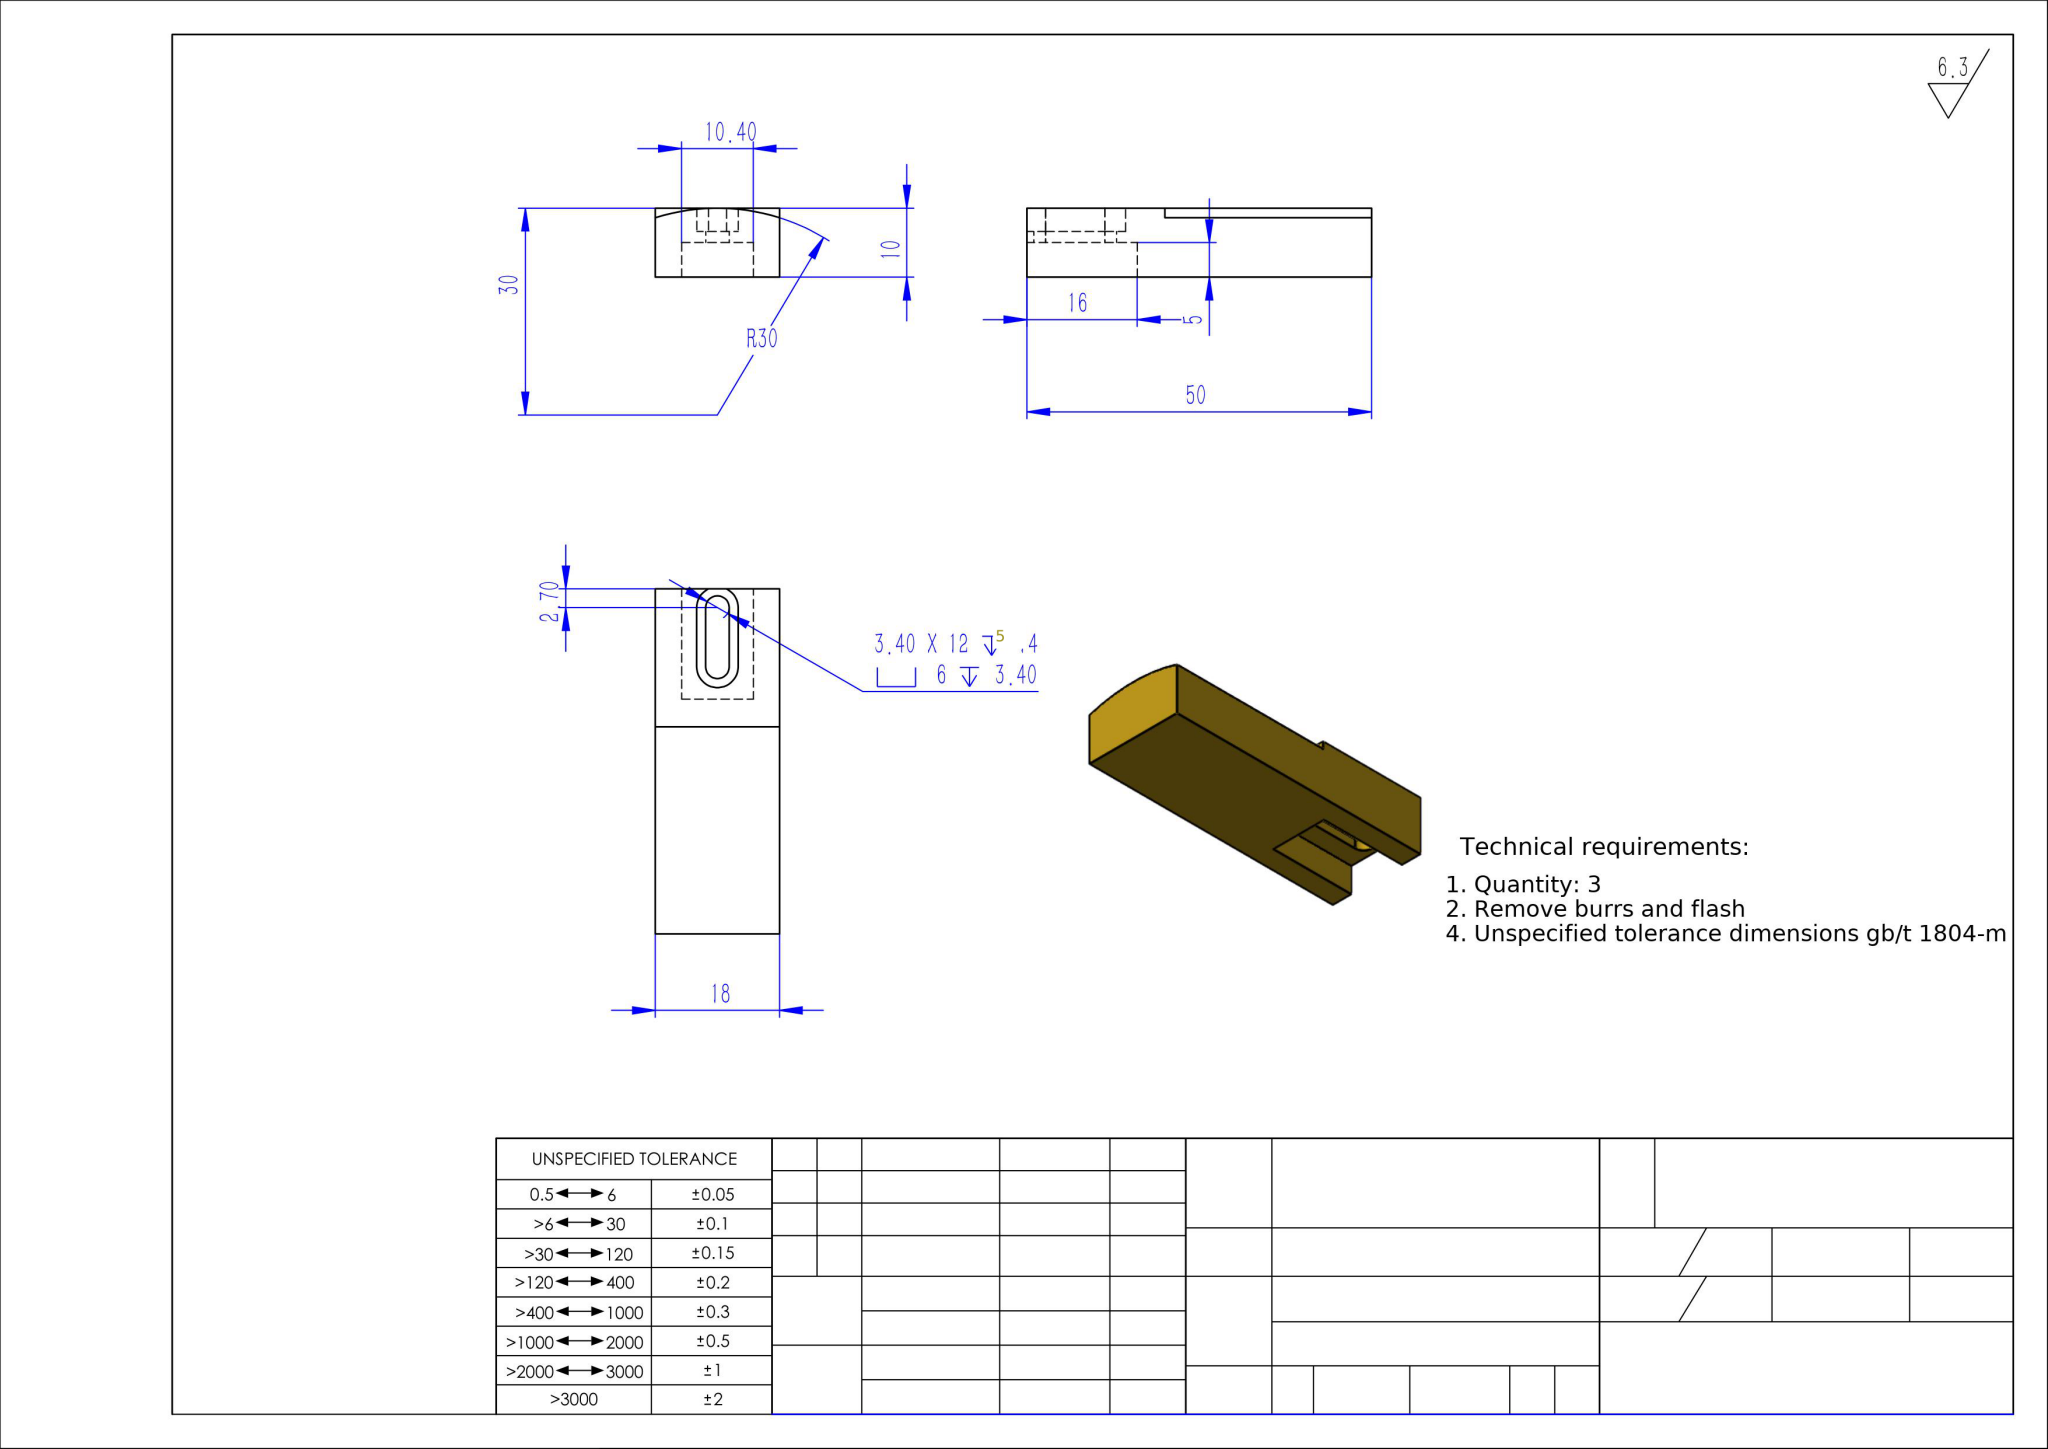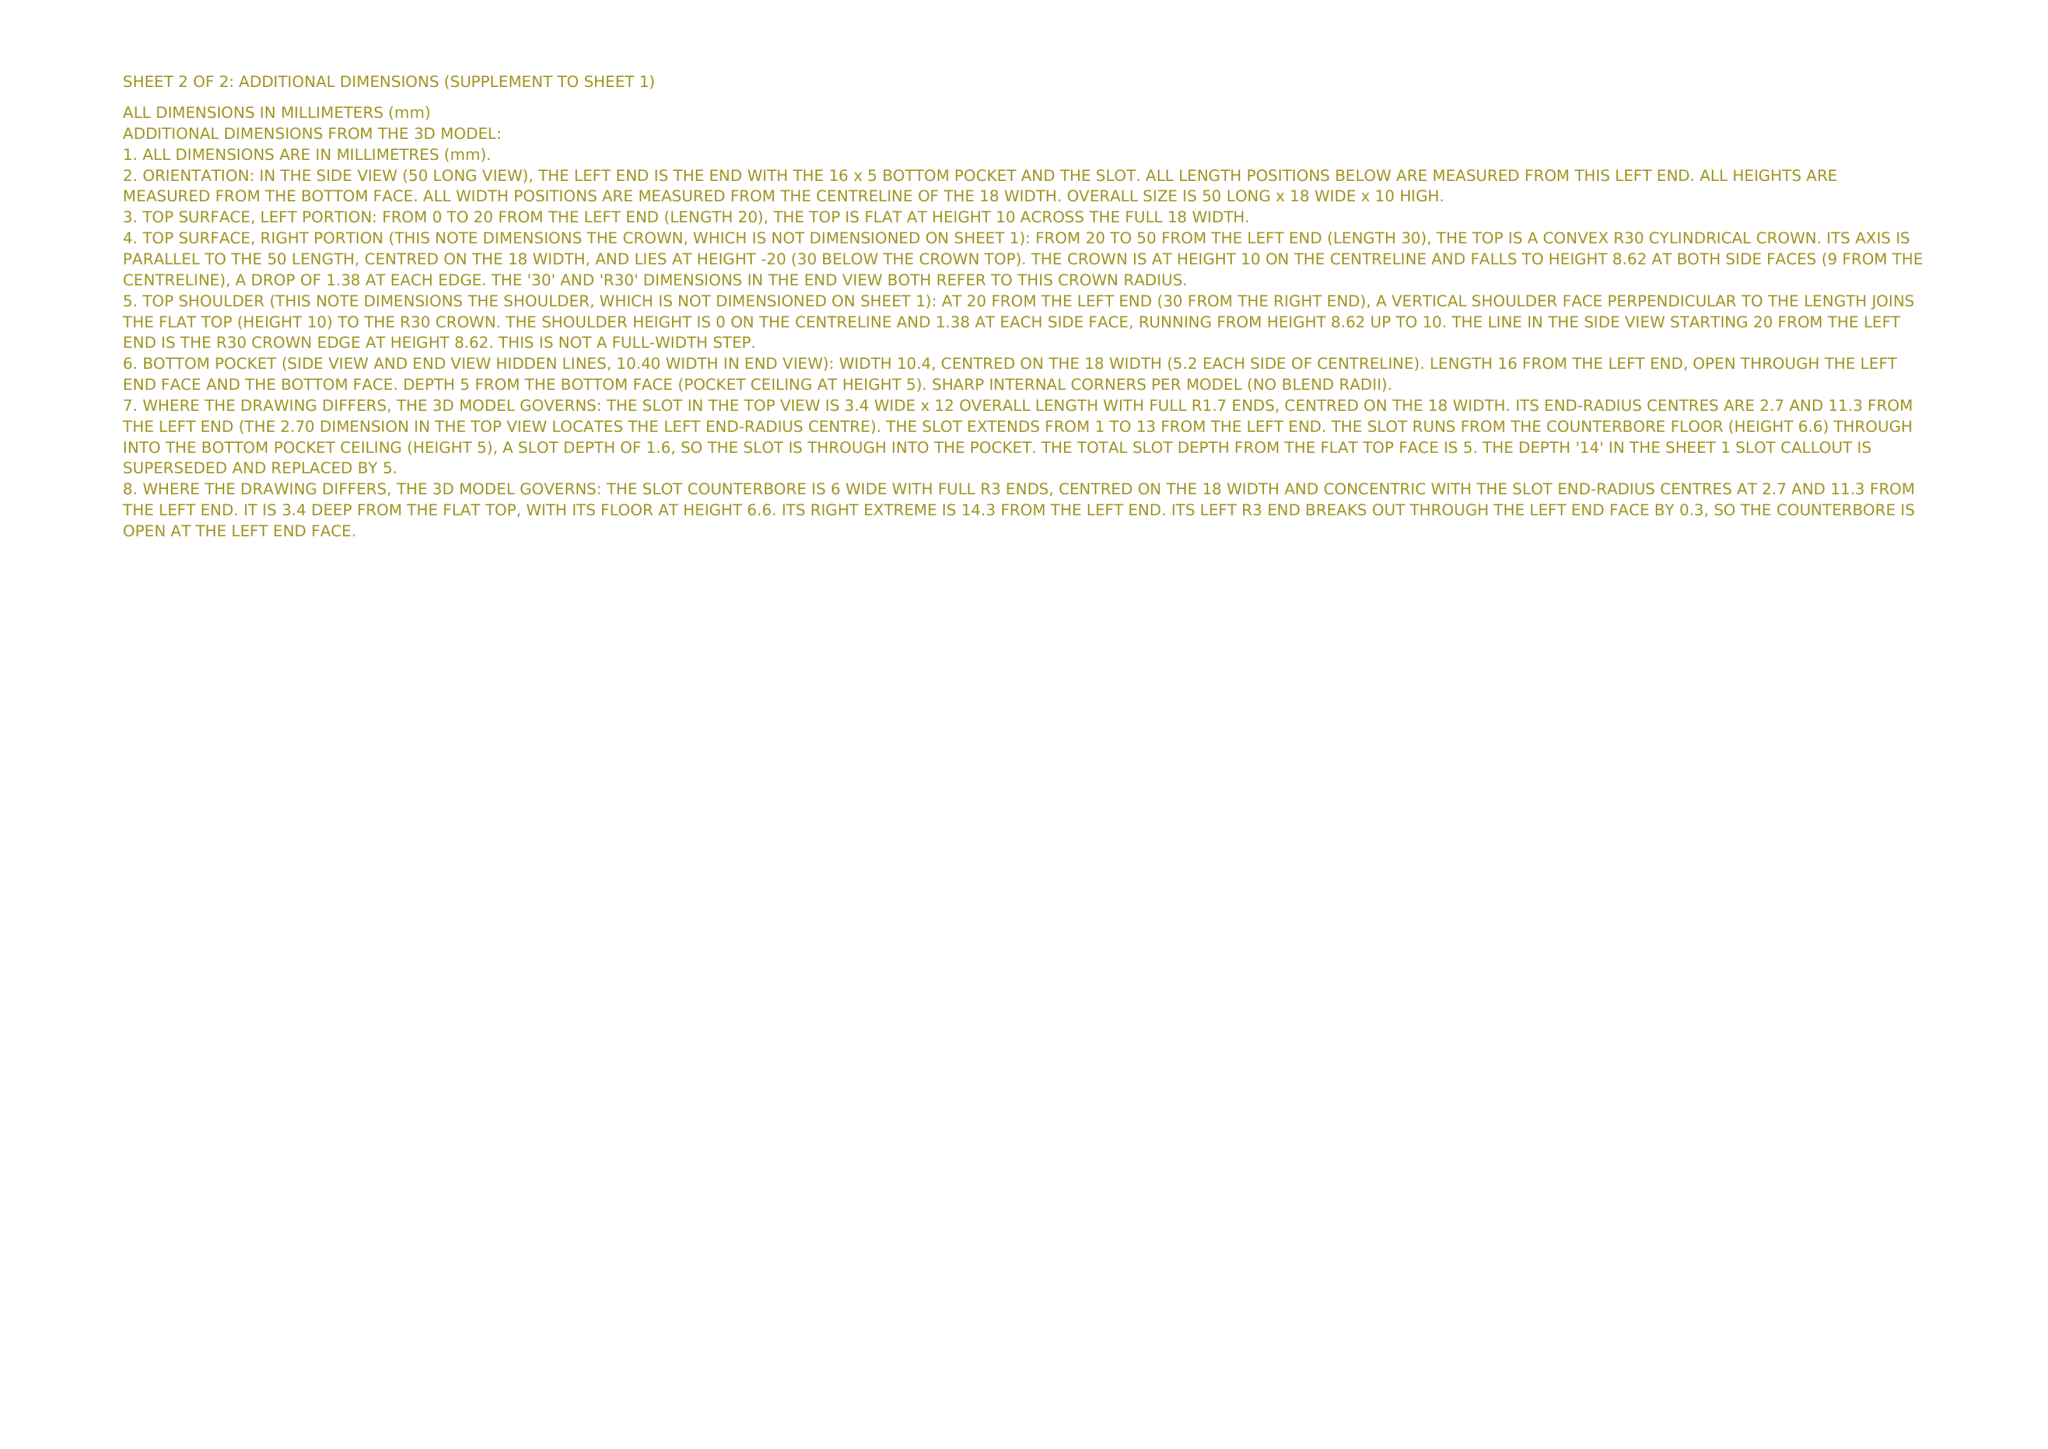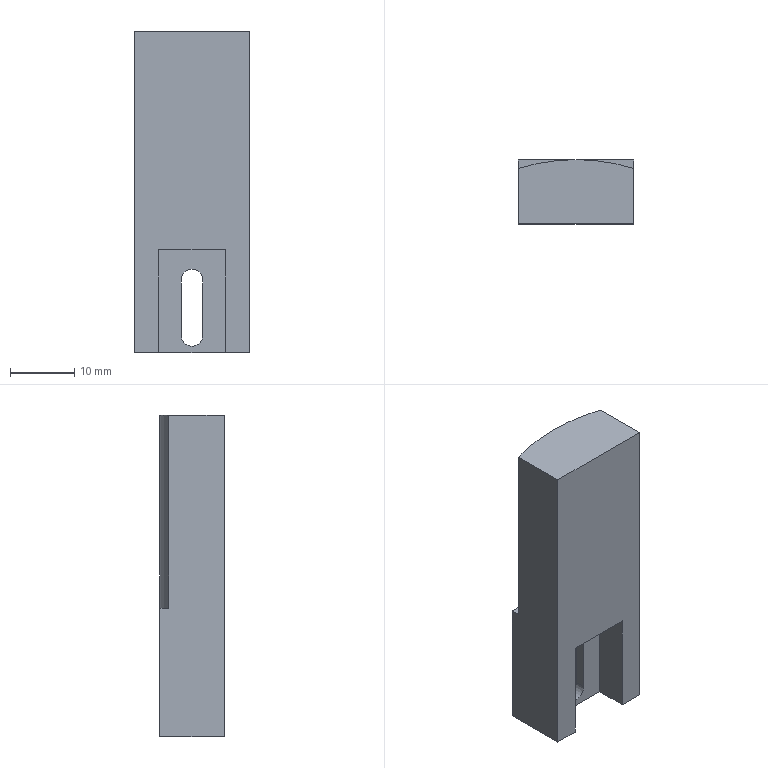Part | NX | mm | Stepped L-Shaped Slotted Mounting Bracket | 1 solid | 25 faces | box 18 x 10 x 50 mm | volume 7591 mm3 | plane 17 | cylinder 8 | commonest cylinder face diameters 6 x4 3.4 x3 60 x1
STEP:
#1=COLOUR_RGB('',0.6471,0.5176,0.);
#2=FILL_AREA_STYLE_COLOUR('',#1);
#3=FILL_AREA_STYLE('',(#2));
#4=SURFACE_STYLE_FILL_AREA(#3);
#5=SURFACE_SIDE_STYLE('',(#4));
#6=SURFACE_STYLE_USAGE(.BOTH.,#5);
#7=PRESENTATION_STYLE_ASSIGNMENT((#6));
#8=CARTESIAN_POINT('',(0.,6.6,-10.7));
#9=VERTEX_POINT('',#8);
#10=CARTESIAN_POINT('',(3.,6.6,-13.7));
#11=VERTEX_POINT('',#10);
#12=CARTESIAN_POINT('',(0.,6.6,-13.7));
#13=DIRECTION('',(0.,1.,0.));
#14=DIRECTION('',(0.,0.,1.));
#15=AXIS2_PLACEMENT_3D('',#12,#13,#14);
#16=CIRCLE('',#15,3.);
#17=EDGE_CURVE('',#9,#11,#16,.T.);
#18=ORIENTED_EDGE('',*,*,#17,.F.);
#19=CARTESIAN_POINT('',(0.,10.,-10.7));
#20=VERTEX_POINT('',#19);
#21=CARTESIAN_POINT('',(0.,10.,-10.7));
#22=DIRECTION('',(0.,1.,0.));
#23=VECTOR('',#22,1000.);
#24=LINE('',#21,#23);
#25=EDGE_CURVE('',#9,#20,#24,.T.);
#26=ORIENTED_EDGE('',*,*,#25,.T.);
#27=CARTESIAN_POINT('',(3.,10.,-13.7));
#28=VERTEX_POINT('',#27);
#29=CARTESIAN_POINT('',(0.,10.,-13.7));
#30=DIRECTION('',(0.,1.,0.));
#31=DIRECTION('',(0.,0.,1.));
#32=AXIS2_PLACEMENT_3D('',#29,#30,#31);
#33=CIRCLE('',#32,3.);
#34=EDGE_CURVE('',#20,#28,#33,.T.);
#35=ORIENTED_EDGE('',*,*,#34,.T.);
#36=CARTESIAN_POINT('',(3.,6.6,-13.7));
#37=DIRECTION('',(-0.,-1.,0.));
#38=VECTOR('',#37,1000.);
#39=LINE('',#36,#38);
#40=EDGE_CURVE('',#28,#11,#39,.T.);
#41=ORIENTED_EDGE('',*,*,#40,.T.);
#42=EDGE_LOOP('',(#18,#26,#35,#41));
#43=FACE_OUTER_BOUND('',#42,.T.);
#44=CARTESIAN_POINT('',(0.,10.,-13.7));
#45=DIRECTION('',(0.,1.,0.));
#46=DIRECTION('',(0.,0.,1.));
#47=AXIS2_PLACEMENT_3D('',#44,#45,#46);
#48=CYLINDRICAL_SURFACE('',#47,3.);
#49=ADVANCED_FACE('',(#43),#48,.F.);
#50=CARTESIAN_POINT('',(1.7,5.,-13.7));
#51=VERTEX_POINT('',#50);
#52=CARTESIAN_POINT('',(0.,5.,-12.));
#53=VERTEX_POINT('',#52);
#54=CARTESIAN_POINT('',(0.,5.,-13.7));
#55=DIRECTION('',(0.,-1.,0.));
#56=DIRECTION('',(0.,0.,1.));
#57=AXIS2_PLACEMENT_3D('',#54,#55,#56);
#58=CIRCLE('',#57,1.7);
#59=EDGE_CURVE('',#51,#53,#58,.T.);
#60=ORIENTED_EDGE('',*,*,#59,.T.);
#61=CARTESIAN_POINT('',(0.,6.6,-12.));
#62=VERTEX_POINT('',#61);
#63=CARTESIAN_POINT('',(0.,10.,-12.));
#64=DIRECTION('',(0.,1.,0.));
#65=VECTOR('',#64,1000.);
#66=LINE('',#63,#65);
#67=EDGE_CURVE('',#53,#62,#66,.T.);
#68=ORIENTED_EDGE('',*,*,#67,.T.);
#69=CARTESIAN_POINT('',(1.7,6.6,-13.7));
#70=VERTEX_POINT('',#69);
#71=CARTESIAN_POINT('',(0.,6.6,-13.7));
#72=DIRECTION('',(0.,1.,0.));
#73=DIRECTION('',(0.,0.,1.));
#74=AXIS2_PLACEMENT_3D('',#71,#72,#73);
#75=CIRCLE('',#74,1.7);
#76=EDGE_CURVE('',#62,#70,#75,.T.);
#77=ORIENTED_EDGE('',*,*,#76,.T.);
#78=CARTESIAN_POINT('',(1.7,-4.,-13.7));
#79=DIRECTION('',(-0.,-1.,0.));
#80=VECTOR('',#79,1000.);
#81=LINE('',#78,#80);
#82=EDGE_CURVE('',#70,#51,#81,.T.);
#83=ORIENTED_EDGE('',*,*,#82,.T.);
#84=EDGE_LOOP('',(#60,#68,#77,#83));
#85=FACE_OUTER_BOUND('',#84,.T.);
#86=CARTESIAN_POINT('',(0.,10.,-13.7));
#87=DIRECTION('',(0.,1.,0.));
#88=DIRECTION('',(0.,0.,1.));
#89=AXIS2_PLACEMENT_3D('',#86,#87,#88);
#90=CYLINDRICAL_SURFACE('',#89,1.7);
#91=ADVANCED_FACE('',(#85),#90,.F.);
#92=CARTESIAN_POINT('',(9.,8.618,25.));
#93=VERTEX_POINT('',#92);
#94=CARTESIAN_POINT('',(9.,0.,25.));
#95=VERTEX_POINT('',#94);
#96=CARTESIAN_POINT('',(9.,10.,25.));
#97=DIRECTION('',(0.,-1.,0.));
#98=VECTOR('',#97,1000.);
#99=LINE('',#96,#98);
#100=EDGE_CURVE('',#93,#95,#99,.T.);
#101=ORIENTED_EDGE('',*,*,#100,.F.);
#102=CARTESIAN_POINT('',(-9.,8.618,25.));
#103=VERTEX_POINT('',#102);
#104=CARTESIAN_POINT('',(0.,-20.,25.));
#105=DIRECTION('',(0.,0.,1.));
#106=DIRECTION('',(1.,0.,0.));
#107=AXIS2_PLACEMENT_3D('',#104,#105,#106);
#108=CIRCLE('',#107,30.);
#109=EDGE_CURVE('',#93,#103,#108,.T.);
#110=ORIENTED_EDGE('',*,*,#109,.T.);
#111=CARTESIAN_POINT('',(-9.,0.,25.));
#112=VERTEX_POINT('',#111);
#113=CARTESIAN_POINT('',(-9.,10.,25.));
#114=DIRECTION('',(0.,-1.,0.));
#115=VECTOR('',#114,1000.);
#116=LINE('',#113,#115);
#117=EDGE_CURVE('',#103,#112,#116,.T.);
#118=ORIENTED_EDGE('',*,*,#117,.T.);
#119=CARTESIAN_POINT('',(-9.,0.,25.));
#120=DIRECTION('',(1.,0.,0.));
#121=VECTOR('',#120,1000.);
#122=LINE('',#119,#121);
#123=EDGE_CURVE('',#112,#95,#122,.T.);
#124=ORIENTED_EDGE('',*,*,#123,.T.);
#125=EDGE_LOOP('',(#101,#110,#118,#124));
#126=FACE_OUTER_BOUND('',#125,.T.);
#127=CARTESIAN_POINT('',(-9.,10.,25.));
#128=DIRECTION('',(0.,0.,-1.));
#129=DIRECTION('',(-1.,0.,0.));
#130=AXIS2_PLACEMENT_3D('',#127,#128,#129);
#131=PLANE('',#130);
#132=ADVANCED_FACE('',(#126),#131,.F.);
#133=CARTESIAN_POINT('',(0.,10.,-5.));
#134=VERTEX_POINT('',#133);
#135=CARTESIAN_POINT('',(-9.,10.,-5.));
#136=VERTEX_POINT('',#135);
#137=CARTESIAN_POINT('',(0.,10.,-5.));
#138=DIRECTION('',(-1.,0.,0.));
#139=VECTOR('',#138,1000.);
#140=LINE('',#137,#139);
#141=EDGE_CURVE('',#134,#136,#140,.T.);
#142=ORIENTED_EDGE('',*,*,#141,.F.);
#143=CARTESIAN_POINT('',(9.,10.,-5.));
#144=VERTEX_POINT('',#143);
#145=CARTESIAN_POINT('',(0.,10.,-5.));
#146=DIRECTION('',(-1.,0.,0.));
#147=VECTOR('',#146,1000.);
#148=LINE('',#145,#147);
#149=EDGE_CURVE('',#144,#134,#148,.T.);
#150=ORIENTED_EDGE('',*,*,#149,.F.);
#151=CARTESIAN_POINT('',(9.,10.,-25.));
#152=VERTEX_POINT('',#151);
#153=CARTESIAN_POINT('',(9.,10.,-25.));
#154=DIRECTION('',(-0.,0.,-1.));
#155=VECTOR('',#154,1000.);
#156=LINE('',#153,#155);
#157=EDGE_CURVE('',#144,#152,#156,.T.);
#158=ORIENTED_EDGE('',*,*,#157,.T.);
#159=CARTESIAN_POINT('',(1.308,10.,-25.));
#160=VERTEX_POINT('',#159);
#161=CARTESIAN_POINT('',(-9.,10.,-25.));
#162=DIRECTION('',(-1.,0.,0.));
#163=VECTOR('',#162,1000.);
#164=LINE('',#161,#163);
#165=EDGE_CURVE('',#152,#160,#164,.T.);
#166=ORIENTED_EDGE('',*,*,#165,.T.);
#167=CARTESIAN_POINT('',(3.,10.,-22.3));
#168=VERTEX_POINT('',#167);
#169=CARTESIAN_POINT('',(0.,10.,-22.3));
#170=DIRECTION('',(0.,1.,0.));
#171=DIRECTION('',(0.,0.,1.));
#172=AXIS2_PLACEMENT_3D('',#169,#170,#171);
#173=CIRCLE('',#172,3.);
#174=EDGE_CURVE('',#168,#160,#173,.T.);
#175=ORIENTED_EDGE('',*,*,#174,.F.);
#176=CARTESIAN_POINT('',(3.,10.,-22.3));
#177=DIRECTION('',(0.,0.,1.));
#178=VECTOR('',#177,1000.);
#179=LINE('',#176,#178);
#180=EDGE_CURVE('',#168,#28,#179,.T.);
#181=ORIENTED_EDGE('',*,*,#180,.T.);
#182=ORIENTED_EDGE('',*,*,#34,.F.);
#183=CARTESIAN_POINT('',(-3.,10.,-13.7));
#184=VERTEX_POINT('',#183);
#185=CARTESIAN_POINT('',(0.,10.,-13.7));
#186=DIRECTION('',(0.,1.,0.));
#187=DIRECTION('',(0.,0.,1.));
#188=AXIS2_PLACEMENT_3D('',#185,#186,#187);
#189=CIRCLE('',#188,3.);
#190=EDGE_CURVE('',#184,#20,#189,.T.);
#191=ORIENTED_EDGE('',*,*,#190,.F.);
#192=CARTESIAN_POINT('',(-3.,10.,-22.3));
#193=VERTEX_POINT('',#192);
#194=CARTESIAN_POINT('',(-3.,10.,-22.3));
#195=DIRECTION('',(0.,0.,1.));
#196=VECTOR('',#195,1000.);
#197=LINE('',#194,#196);
#198=EDGE_CURVE('',#193,#184,#197,.T.);
#199=ORIENTED_EDGE('',*,*,#198,.F.);
#200=CARTESIAN_POINT('',(-1.308,10.,-25.));
#201=VERTEX_POINT('',#200);
#202=CARTESIAN_POINT('',(0.,10.,-22.3));
#203=DIRECTION('',(0.,1.,0.));
#204=DIRECTION('',(0.,0.,1.));
#205=AXIS2_PLACEMENT_3D('',#202,#203,#204);
#206=CIRCLE('',#205,3.);
#207=EDGE_CURVE('',#201,#193,#206,.T.);
#208=ORIENTED_EDGE('',*,*,#207,.F.);
#209=CARTESIAN_POINT('',(-9.,10.,-25.));
#210=VERTEX_POINT('',#209);
#211=CARTESIAN_POINT('',(-9.,10.,-25.));
#212=DIRECTION('',(-1.,0.,0.));
#213=VECTOR('',#212,1000.);
#214=LINE('',#211,#213);
#215=EDGE_CURVE('',#201,#210,#214,.T.);
#216=ORIENTED_EDGE('',*,*,#215,.T.);
#217=CARTESIAN_POINT('',(-9.,10.,-25.));
#218=DIRECTION('',(0.,0.,1.));
#219=VECTOR('',#218,1000.);
#220=LINE('',#217,#219);
#221=EDGE_CURVE('',#210,#136,#220,.T.);
#222=ORIENTED_EDGE('',*,*,#221,.T.);
#223=EDGE_LOOP('',(#142,#150,#158,#166,#175,#181,#182,#191,#199,#208,#216,#222));
#224=FACE_OUTER_BOUND('',#223,.T.);
#225=CARTESIAN_POINT('',(0.,10.,0.));
#226=DIRECTION('',(0.,1.,0.));
#227=DIRECTION('',(0.,0.,1.));
#228=AXIS2_PLACEMENT_3D('',#225,#226,#227);
#229=PLANE('',#228);
#230=ADVANCED_FACE('',(#224),#229,.T.);
#231=CARTESIAN_POINT('',(9.,8.618,-5.));
#232=VERTEX_POINT('',#231);
#233=CARTESIAN_POINT('',(9.,8.618,-5.));
#234=DIRECTION('',(0.,0.,1.));
#235=VECTOR('',#234,1000.);
#236=LINE('',#233,#235);
#237=EDGE_CURVE('',#232,#93,#236,.T.);
#238=ORIENTED_EDGE('',*,*,#237,.T.);
#239=ORIENTED_EDGE('',*,*,#100,.T.);
#240=CARTESIAN_POINT('',(9.,0.,-25.));
#241=VERTEX_POINT('',#240);
#242=CARTESIAN_POINT('',(9.,0.,-25.));
#243=DIRECTION('',(-0.,0.,-1.));
#244=VECTOR('',#243,1000.);
#245=LINE('',#242,#244);
#246=EDGE_CURVE('',#95,#241,#245,.T.);
#247=ORIENTED_EDGE('',*,*,#246,.T.);
#248=CARTESIAN_POINT('',(9.,10.,-25.));
#249=DIRECTION('',(0.,-1.,0.));
#250=VECTOR('',#249,1000.);
#251=LINE('',#248,#250);
#252=EDGE_CURVE('',#152,#241,#251,.T.);
#253=ORIENTED_EDGE('',*,*,#252,.F.);
#254=ORIENTED_EDGE('',*,*,#157,.F.);
#255=CARTESIAN_POINT('',(9.,0.,-5.));
#256=DIRECTION('',(0.,1.,0.));
#257=VECTOR('',#256,1000.);
#258=LINE('',#255,#257);
#259=EDGE_CURVE('',#232,#144,#258,.T.);
#260=ORIENTED_EDGE('',*,*,#259,.F.);
#261=EDGE_LOOP('',(#238,#239,#247,#253,#254,#260));
#262=FACE_OUTER_BOUND('',#261,.T.);
#263=CARTESIAN_POINT('',(9.,10.,-25.));
#264=DIRECTION('',(-1.,0.,0.));
#265=DIRECTION('',(0.,0.,1.));
#266=AXIS2_PLACEMENT_3D('',#263,#264,#265);
#267=PLANE('',#266);
#268=ADVANCED_FACE('',(#262),#267,.F.);
#269=CARTESIAN_POINT('',(-9.,8.618,-5.));
#270=VERTEX_POINT('',#269);
#271=CARTESIAN_POINT('',(-9.,8.618,-5.));
#272=DIRECTION('',(0.,0.,1.));
#273=VECTOR('',#272,1000.);
#274=LINE('',#271,#273);
#275=EDGE_CURVE('',#270,#103,#274,.T.);
#276=ORIENTED_EDGE('',*,*,#275,.F.);
#277=CARTESIAN_POINT('',(-9.,0.,-5.));
#278=DIRECTION('',(0.,-1.,0.));
#279=VECTOR('',#278,1000.);
#280=LINE('',#277,#279);
#281=EDGE_CURVE('',#136,#270,#280,.T.);
#282=ORIENTED_EDGE('',*,*,#281,.F.);
#283=ORIENTED_EDGE('',*,*,#221,.F.);
#284=CARTESIAN_POINT('',(-9.,0.,-25.));
#285=VERTEX_POINT('',#284);
#286=CARTESIAN_POINT('',(-9.,10.,-25.));
#287=DIRECTION('',(0.,-1.,0.));
#288=VECTOR('',#287,1000.);
#289=LINE('',#286,#288);
#290=EDGE_CURVE('',#210,#285,#289,.T.);
#291=ORIENTED_EDGE('',*,*,#290,.T.);
#292=CARTESIAN_POINT('',(-9.,0.,-25.));
#293=DIRECTION('',(0.,0.,1.));
#294=VECTOR('',#293,1000.);
#295=LINE('',#292,#294);
#296=EDGE_CURVE('',#285,#112,#295,.T.);
#297=ORIENTED_EDGE('',*,*,#296,.T.);
#298=ORIENTED_EDGE('',*,*,#117,.F.);
#299=EDGE_LOOP('',(#276,#282,#283,#291,#297,#298));
#300=FACE_OUTER_BOUND('',#299,.T.);
#301=CARTESIAN_POINT('',(-9.,10.,-25.));
#302=DIRECTION('',(1.,0.,-0.));
#303=DIRECTION('',(-0.,0.,-1.));
#304=AXIS2_PLACEMENT_3D('',#301,#302,#303);
#305=PLANE('',#304);
#306=ADVANCED_FACE('',(#300),#305,.F.);
#307=CARTESIAN_POINT('',(-5.2,0.,-25.));
#308=VERTEX_POINT('',#307);
#309=CARTESIAN_POINT('',(-9.,0.,-25.));
#310=DIRECTION('',(-1.,0.,0.));
#311=VECTOR('',#310,1000.);
#312=LINE('',#309,#311);
#313=EDGE_CURVE('',#308,#285,#312,.T.);
#314=ORIENTED_EDGE('',*,*,#313,.F.);
#315=CARTESIAN_POINT('',(-5.2,0.,-9.));
#316=VERTEX_POINT('',#315);
#317=CARTESIAN_POINT('',(-5.2,0.,-25.));
#318=DIRECTION('',(0.,0.,-1.));
#319=VECTOR('',#318,1000.);
#320=LINE('',#317,#319);
#321=EDGE_CURVE('',#316,#308,#320,.T.);
#322=ORIENTED_EDGE('',*,*,#321,.F.);
#323=CARTESIAN_POINT('',(5.2,0.,-9.));
#324=VERTEX_POINT('',#323);
#325=CARTESIAN_POINT('',(-5.2,0.,-9.));
#326=DIRECTION('',(-1.,0.,0.));
#327=VECTOR('',#326,1000.);
#328=LINE('',#325,#327);
#329=EDGE_CURVE('',#324,#316,#328,.T.);
#330=ORIENTED_EDGE('',*,*,#329,.F.);
#331=CARTESIAN_POINT('',(5.2,0.,-25.));
#332=VERTEX_POINT('',#331);
#333=CARTESIAN_POINT('',(5.2,0.,-25.));
#334=DIRECTION('',(0.,0.,1.));
#335=VECTOR('',#334,1000.);
#336=LINE('',#333,#335);
#337=EDGE_CURVE('',#332,#324,#336,.T.);
#338=ORIENTED_EDGE('',*,*,#337,.F.);
#339=CARTESIAN_POINT('',(-9.,0.,-25.));
#340=DIRECTION('',(-1.,0.,0.));
#341=VECTOR('',#340,1000.);
#342=LINE('',#339,#341);
#343=EDGE_CURVE('',#241,#332,#342,.T.);
#344=ORIENTED_EDGE('',*,*,#343,.F.);
#345=ORIENTED_EDGE('',*,*,#246,.F.);
#346=ORIENTED_EDGE('',*,*,#123,.F.);
#347=ORIENTED_EDGE('',*,*,#296,.F.);
#348=EDGE_LOOP('',(#314,#322,#330,#338,#344,#345,#346,#347));
#349=FACE_OUTER_BOUND('',#348,.T.);
#350=CARTESIAN_POINT('',(0.,0.,0.));
#351=DIRECTION('',(0.,1.,0.));
#352=DIRECTION('',(0.,0.,1.));
#353=AXIS2_PLACEMENT_3D('',#350,#351,#352);
#354=PLANE('',#353);
#355=ADVANCED_FACE('',(#349),#354,.F.);
#356=CARTESIAN_POINT('',(-5.2,5.,-25.));
#357=VERTEX_POINT('',#356);
#358=CARTESIAN_POINT('',(5.2,5.,-25.));
#359=VERTEX_POINT('',#358);
#360=CARTESIAN_POINT('',(-5.2,5.,-25.));
#361=DIRECTION('',(1.,0.,0.));
#362=VECTOR('',#361,1000.);
#363=LINE('',#360,#362);
#364=EDGE_CURVE('',#357,#359,#363,.T.);
#365=ORIENTED_EDGE('',*,*,#364,.F.);
#366=CARTESIAN_POINT('',(-5.2,5.,-25.));
#367=DIRECTION('',(0.,-1.,0.));
#368=VECTOR('',#367,1000.);
#369=LINE('',#366,#368);
#370=EDGE_CURVE('',#357,#308,#369,.T.);
#371=ORIENTED_EDGE('',*,*,#370,.T.);
#372=ORIENTED_EDGE('',*,*,#313,.T.);
#373=ORIENTED_EDGE('',*,*,#290,.F.);
#374=ORIENTED_EDGE('',*,*,#215,.F.);
#375=CARTESIAN_POINT('',(-1.308,6.6,-25.));
#376=VERTEX_POINT('',#375);
#377=CARTESIAN_POINT('',(-1.308,10.,-25.));
#378=DIRECTION('',(0.,-1.,0.));
#379=VECTOR('',#378,1000.);
#380=LINE('',#377,#379);
#381=EDGE_CURVE('',#201,#376,#380,.T.);
#382=ORIENTED_EDGE('',*,*,#381,.T.);
#383=CARTESIAN_POINT('',(1.308,6.6,-25.));
#384=VERTEX_POINT('',#383);
#385=CARTESIAN_POINT('',(-9.,6.6,-25.));
#386=DIRECTION('',(1.,0.,0.));
#387=VECTOR('',#386,1000.);
#388=LINE('',#385,#387);
#389=EDGE_CURVE('',#376,#384,#388,.T.);
#390=ORIENTED_EDGE('',*,*,#389,.T.);
#391=CARTESIAN_POINT('',(1.308,10.,-25.));
#392=DIRECTION('',(0.,1.,0.));
#393=VECTOR('',#392,1000.);
#394=LINE('',#391,#393);
#395=EDGE_CURVE('',#384,#160,#394,.T.);
#396=ORIENTED_EDGE('',*,*,#395,.T.);
#397=ORIENTED_EDGE('',*,*,#165,.F.);
#398=ORIENTED_EDGE('',*,*,#252,.T.);
#399=ORIENTED_EDGE('',*,*,#343,.T.);
#400=CARTESIAN_POINT('',(5.2,5.,-25.));
#401=DIRECTION('',(0.,-1.,0.));
#402=VECTOR('',#401,1000.);
#403=LINE('',#400,#402);
#404=EDGE_CURVE('',#359,#332,#403,.T.);
#405=ORIENTED_EDGE('',*,*,#404,.F.);
#406=EDGE_LOOP('',(#365,#371,#372,#373,#374,#382,#390,#396,#397,#398,#399,#405));
#407=FACE_OUTER_BOUND('',#406,.T.);
#408=CARTESIAN_POINT('',(-9.,10.,-25.));
#409=DIRECTION('',(0.,0.,1.));
#410=DIRECTION('',(1.,0.,0.));
#411=AXIS2_PLACEMENT_3D('',#408,#409,#410);
#412=PLANE('',#411);
#413=ADVANCED_FACE('',(#407),#412,.F.);
#414=CARTESIAN_POINT('',(-1.7,5.,-22.3));
#415=VERTEX_POINT('',#414);
#416=CARTESIAN_POINT('',(-1.7,6.6,-22.3));
#417=VERTEX_POINT('',#416);
#418=CARTESIAN_POINT('',(-1.7,10.,-22.3));
#419=DIRECTION('',(0.,1.,0.));
#420=VECTOR('',#419,1000.);
#421=LINE('',#418,#420);
#422=EDGE_CURVE('',#415,#417,#421,.T.);
#423=ORIENTED_EDGE('',*,*,#422,.F.);
#424=CARTESIAN_POINT('',(1.7,5.,-22.3));
#425=VERTEX_POINT('',#424);
#426=CARTESIAN_POINT('',(0.,5.,-22.3));
#427=DIRECTION('',(0.,-1.,0.));
#428=DIRECTION('',(0.,0.,1.));
#429=AXIS2_PLACEMENT_3D('',#426,#427,#428);
#430=CIRCLE('',#429,1.7);
#431=EDGE_CURVE('',#415,#425,#430,.T.);
#432=ORIENTED_EDGE('',*,*,#431,.T.);
#433=CARTESIAN_POINT('',(1.7,6.6,-22.3));
#434=VERTEX_POINT('',#433);
#435=CARTESIAN_POINT('',(1.7,-4.,-22.3));
#436=DIRECTION('',(-0.,-1.,0.));
#437=VECTOR('',#436,1000.);
#438=LINE('',#435,#437);
#439=EDGE_CURVE('',#434,#425,#438,.T.);
#440=ORIENTED_EDGE('',*,*,#439,.F.);
#441=CARTESIAN_POINT('',(0.,6.6,-22.3));
#442=DIRECTION('',(0.,1.,0.));
#443=DIRECTION('',(0.,0.,1.));
#444=AXIS2_PLACEMENT_3D('',#441,#442,#443);
#445=CIRCLE('',#444,1.7);
#446=EDGE_CURVE('',#434,#417,#445,.T.);
#447=ORIENTED_EDGE('',*,*,#446,.T.);
#448=EDGE_LOOP('',(#423,#432,#440,#447));
#449=FACE_OUTER_BOUND('',#448,.T.);
#450=CARTESIAN_POINT('',(0.,10.,-22.3));
#451=DIRECTION('',(0.,1.,0.));
#452=DIRECTION('',(0.,0.,1.));
#453=AXIS2_PLACEMENT_3D('',#450,#451,#452);
#454=CYLINDRICAL_SURFACE('',#453,1.7);
#455=ADVANCED_FACE('',(#449),#454,.F.);
#456=ORIENTED_EDGE('',*,*,#67,.F.);
#457=CARTESIAN_POINT('',(-1.7,5.,-13.7));
#458=VERTEX_POINT('',#457);
#459=CARTESIAN_POINT('',(0.,5.,-13.7));
#460=DIRECTION('',(0.,-1.,0.));
#461=DIRECTION('',(0.,0.,1.));
#462=AXIS2_PLACEMENT_3D('',#459,#460,#461);
#463=CIRCLE('',#462,1.7);
#464=EDGE_CURVE('',#53,#458,#463,.T.);
#465=ORIENTED_EDGE('',*,*,#464,.T.);
#466=CARTESIAN_POINT('',(-1.7,6.6,-13.7));
#467=VERTEX_POINT('',#466);
#468=CARTESIAN_POINT('',(-1.7,10.,-13.7));
#469=DIRECTION('',(0.,-1.,0.));
#470=VECTOR('',#469,1000.);
#471=LINE('',#468,#470);
#472=EDGE_CURVE('',#467,#458,#471,.T.);
#473=ORIENTED_EDGE('',*,*,#472,.F.);
#474=CARTESIAN_POINT('',(0.,6.6,-13.7));
#475=DIRECTION('',(0.,1.,0.));
#476=DIRECTION('',(0.,0.,1.));
#477=AXIS2_PLACEMENT_3D('',#474,#475,#476);
#478=CIRCLE('',#477,1.7);
#479=EDGE_CURVE('',#467,#62,#478,.T.);
#480=ORIENTED_EDGE('',*,*,#479,.T.);
#481=EDGE_LOOP('',(#456,#465,#473,#480));
#482=FACE_OUTER_BOUND('',#481,.T.);
#483=CARTESIAN_POINT('',(0.,10.,-13.7));
#484=DIRECTION('',(0.,1.,0.));
#485=DIRECTION('',(0.,0.,1.));
#486=AXIS2_PLACEMENT_3D('',#483,#484,#485);
#487=CYLINDRICAL_SURFACE('',#486,1.7);
#488=ADVANCED_FACE('',(#482),#487,.F.);
#489=CARTESIAN_POINT('',(1.7,5.,-22.3));
#490=DIRECTION('',(0.,0.,-1.));
#491=VECTOR('',#490,1000.);
#492=LINE('',#489,#491);
#493=EDGE_CURVE('',#51,#425,#492,.T.);
#494=ORIENTED_EDGE('',*,*,#493,.F.);
#495=ORIENTED_EDGE('',*,*,#82,.F.);
#496=CARTESIAN_POINT('',(1.7,6.6,-22.3));
#497=DIRECTION('',(0.,0.,1.));
#498=VECTOR('',#497,1000.);
#499=LINE('',#496,#498);
#500=EDGE_CURVE('',#434,#70,#499,.T.);
#501=ORIENTED_EDGE('',*,*,#500,.F.);
#502=ORIENTED_EDGE('',*,*,#439,.T.);
#503=EDGE_LOOP('',(#494,#495,#501,#502));
#504=FACE_OUTER_BOUND('',#503,.T.);
#505=CARTESIAN_POINT('',(1.7,-4.,-22.3));
#506=DIRECTION('',(-1.,0.,0.));
#507=DIRECTION('',(-0.,-1.,0.));
#508=AXIS2_PLACEMENT_3D('',#505,#506,#507);
#509=PLANE('',#508);
#510=ADVANCED_FACE('',(#504),#509,.T.);
#511=ORIENTED_EDGE('',*,*,#472,.T.);
#512=CARTESIAN_POINT('',(-1.7,5.,-22.3));
#513=DIRECTION('',(0.,0.,-1.));
#514=VECTOR('',#513,1000.);
#515=LINE('',#512,#514);
#516=EDGE_CURVE('',#458,#415,#515,.T.);
#517=ORIENTED_EDGE('',*,*,#516,.T.);
#518=ORIENTED_EDGE('',*,*,#422,.T.);
#519=CARTESIAN_POINT('',(-1.7,6.6,-22.3));
#520=DIRECTION('',(0.,0.,1.));
#521=VECTOR('',#520,1000.);
#522=LINE('',#519,#521);
#523=EDGE_CURVE('',#417,#467,#522,.T.);
#524=ORIENTED_EDGE('',*,*,#523,.T.);
#525=EDGE_LOOP('',(#511,#517,#518,#524));
#526=FACE_OUTER_BOUND('',#525,.T.);
#527=CARTESIAN_POINT('',(-1.7,10.,-22.3));
#528=DIRECTION('',(-1.,0.,0.));
#529=DIRECTION('',(0.,0.,1.));
#530=AXIS2_PLACEMENT_3D('',#527,#528,#529);
#531=PLANE('',#530);
#532=ADVANCED_FACE('',(#526),#531,.F.);
#533=ORIENTED_EDGE('',*,*,#479,.F.);
#534=ORIENTED_EDGE('',*,*,#523,.F.);
#535=ORIENTED_EDGE('',*,*,#446,.F.);
#536=ORIENTED_EDGE('',*,*,#500,.T.);
#537=ORIENTED_EDGE('',*,*,#76,.F.);
#538=EDGE_LOOP('',(#533,#534,#535,#536,#537));
#539=FACE_BOUND('',#538,.T.);
#540=CARTESIAN_POINT('',(-3.,6.6,-22.3));
#541=VERTEX_POINT('',#540);
#542=CARTESIAN_POINT('',(0.,6.6,-22.3));
#543=DIRECTION('',(0.,1.,0.));
#544=DIRECTION('',(0.,0.,1.));
#545=AXIS2_PLACEMENT_3D('',#542,#543,#544);
#546=CIRCLE('',#545,3.);
#547=EDGE_CURVE('',#376,#541,#546,.T.);
#548=ORIENTED_EDGE('',*,*,#547,.T.);
#549=CARTESIAN_POINT('',(-3.,6.6,-13.7));
#550=VERTEX_POINT('',#549);
#551=CARTESIAN_POINT('',(-3.,6.6,-22.3));
#552=DIRECTION('',(0.,0.,1.));
#553=VECTOR('',#552,1000.);
#554=LINE('',#551,#553);
#555=EDGE_CURVE('',#541,#550,#554,.T.);
#556=ORIENTED_EDGE('',*,*,#555,.T.);
#557=CARTESIAN_POINT('',(0.,6.6,-13.7));
#558=DIRECTION('',(0.,1.,0.));
#559=DIRECTION('',(0.,0.,1.));
#560=AXIS2_PLACEMENT_3D('',#557,#558,#559);
#561=CIRCLE('',#560,3.);
#562=EDGE_CURVE('',#550,#9,#561,.T.);
#563=ORIENTED_EDGE('',*,*,#562,.T.);
#564=ORIENTED_EDGE('',*,*,#17,.T.);
#565=CARTESIAN_POINT('',(3.,6.6,-22.3));
#566=VERTEX_POINT('',#565);
#567=CARTESIAN_POINT('',(3.,6.6,-22.3));
#568=DIRECTION('',(0.,0.,1.));
#569=VECTOR('',#568,1000.);
#570=LINE('',#567,#569);
#571=EDGE_CURVE('',#566,#11,#570,.T.);
#572=ORIENTED_EDGE('',*,*,#571,.F.);
#573=CARTESIAN_POINT('',(0.,6.6,-22.3));
#574=DIRECTION('',(0.,1.,0.));
#575=DIRECTION('',(0.,0.,1.));
#576=AXIS2_PLACEMENT_3D('',#573,#574,#575);
#577=CIRCLE('',#576,3.);
#578=EDGE_CURVE('',#566,#384,#577,.T.);
#579=ORIENTED_EDGE('',*,*,#578,.T.);
#580=ORIENTED_EDGE('',*,*,#389,.F.);
#581=EDGE_LOOP('',(#548,#556,#563,#564,#572,#579,#580));
#582=FACE_OUTER_BOUND('',#581,.T.);
#583=CARTESIAN_POINT('',(1.7,6.6,-13.7));
#584=DIRECTION('',(0.,-1.,0.));
#585=DIRECTION('',(0.,0.,-1.));
#586=AXIS2_PLACEMENT_3D('',#583,#584,#585);
#587=PLANE('',#586);
#588=ADVANCED_FACE('',(#539,#582),#587,.F.);
#589=ORIENTED_EDGE('',*,*,#578,.F.);
#590=CARTESIAN_POINT('',(3.,6.6,-22.3));
#591=DIRECTION('',(-0.,-1.,0.));
#592=VECTOR('',#591,1000.);
#593=LINE('',#590,#592);
#594=EDGE_CURVE('',#168,#566,#593,.T.);
#595=ORIENTED_EDGE('',*,*,#594,.F.);
#596=ORIENTED_EDGE('',*,*,#174,.T.);
#597=ORIENTED_EDGE('',*,*,#395,.F.);
#598=EDGE_LOOP('',(#589,#595,#596,#597));
#599=FACE_OUTER_BOUND('',#598,.T.);
#600=CARTESIAN_POINT('',(0.,10.,-22.3));
#601=DIRECTION('',(0.,1.,0.));
#602=DIRECTION('',(0.,0.,1.));
#603=AXIS2_PLACEMENT_3D('',#600,#601,#602);
#604=CYLINDRICAL_SURFACE('',#603,3.);
#605=ADVANCED_FACE('',(#599),#604,.F.);
#606=ORIENTED_EDGE('',*,*,#207,.T.);
#607=CARTESIAN_POINT('',(-3.,10.,-22.3));
#608=DIRECTION('',(0.,1.,0.));
#609=VECTOR('',#608,1000.);
#610=LINE('',#607,#609);
#611=EDGE_CURVE('',#541,#193,#610,.T.);
#612=ORIENTED_EDGE('',*,*,#611,.F.);
#613=ORIENTED_EDGE('',*,*,#547,.F.);
#614=ORIENTED_EDGE('',*,*,#381,.F.);
#615=EDGE_LOOP('',(#606,#612,#613,#614));
#616=FACE_OUTER_BOUND('',#615,.T.);
#617=CARTESIAN_POINT('',(0.,10.,-22.3));
#618=DIRECTION('',(0.,1.,0.));
#619=DIRECTION('',(0.,0.,1.));
#620=AXIS2_PLACEMENT_3D('',#617,#618,#619);
#621=CYLINDRICAL_SURFACE('',#620,3.);
#622=ADVANCED_FACE('',(#616),#621,.F.);
#623=ORIENTED_EDGE('',*,*,#25,.F.);
#624=ORIENTED_EDGE('',*,*,#562,.F.);
#625=CARTESIAN_POINT('',(-3.,10.,-13.7));
#626=DIRECTION('',(0.,-1.,0.));
#627=VECTOR('',#626,1000.);
#628=LINE('',#625,#627);
#629=EDGE_CURVE('',#184,#550,#628,.T.);
#630=ORIENTED_EDGE('',*,*,#629,.F.);
#631=ORIENTED_EDGE('',*,*,#190,.T.);
#632=EDGE_LOOP('',(#623,#624,#630,#631));
#633=FACE_OUTER_BOUND('',#632,.T.);
#634=CARTESIAN_POINT('',(0.,10.,-13.7));
#635=DIRECTION('',(0.,1.,0.));
#636=DIRECTION('',(0.,0.,1.));
#637=AXIS2_PLACEMENT_3D('',#634,#635,#636);
#638=CYLINDRICAL_SURFACE('',#637,3.);
#639=ADVANCED_FACE('',(#633),#638,.F.);
#640=ORIENTED_EDGE('',*,*,#40,.F.);
#641=ORIENTED_EDGE('',*,*,#180,.F.);
#642=ORIENTED_EDGE('',*,*,#594,.T.);
#643=ORIENTED_EDGE('',*,*,#571,.T.);
#644=EDGE_LOOP('',(#640,#641,#642,#643));
#645=FACE_OUTER_BOUND('',#644,.T.);
#646=CARTESIAN_POINT('',(3.,6.6,-22.3));
#647=DIRECTION('',(-1.,0.,0.));
#648=DIRECTION('',(-0.,-1.,0.));
#649=AXIS2_PLACEMENT_3D('',#646,#647,#648);
#650=PLANE('',#649);
#651=ADVANCED_FACE('',(#645),#650,.T.);
#652=ORIENTED_EDGE('',*,*,#629,.T.);
#653=ORIENTED_EDGE('',*,*,#555,.F.);
#654=ORIENTED_EDGE('',*,*,#611,.T.);
#655=ORIENTED_EDGE('',*,*,#198,.T.);
#656=EDGE_LOOP('',(#652,#653,#654,#655));
#657=FACE_OUTER_BOUND('',#656,.T.);
#658=CARTESIAN_POINT('',(-3.,10.,-22.3));
#659=DIRECTION('',(-1.,0.,0.));
#660=DIRECTION('',(0.,0.,1.));
#661=AXIS2_PLACEMENT_3D('',#658,#659,#660);
#662=PLANE('',#661);
#663=ADVANCED_FACE('',(#657),#662,.F.);
#664=ORIENTED_EDGE('',*,*,#321,.T.);
#665=ORIENTED_EDGE('',*,*,#370,.F.);
#666=CARTESIAN_POINT('',(-5.2,5.,-9.));
#667=VERTEX_POINT('',#666);
#668=CARTESIAN_POINT('',(-5.2,5.,-25.));
#669=DIRECTION('',(0.,0.,-1.));
#670=VECTOR('',#669,1000.);
#671=LINE('',#668,#670);
#672=EDGE_CURVE('',#667,#357,#671,.T.);
#673=ORIENTED_EDGE('',*,*,#672,.F.);
#674=CARTESIAN_POINT('',(-5.2,5.,-9.));
#675=DIRECTION('',(0.,-1.,0.));
#676=VECTOR('',#675,1000.);
#677=LINE('',#674,#676);
#678=EDGE_CURVE('',#667,#316,#677,.T.);
#679=ORIENTED_EDGE('',*,*,#678,.T.);
#680=EDGE_LOOP('',(#664,#665,#673,#679));
#681=FACE_OUTER_BOUND('',#680,.T.);
#682=CARTESIAN_POINT('',(-5.2,5.,-25.));
#683=DIRECTION('',(-1.,0.,0.));
#684=DIRECTION('',(0.,0.,1.));
#685=AXIS2_PLACEMENT_3D('',#682,#683,#684);
#686=PLANE('',#685);
#687=ADVANCED_FACE('',(#681),#686,.F.);
#688=ORIENTED_EDGE('',*,*,#329,.T.);
#689=ORIENTED_EDGE('',*,*,#678,.F.);
#690=CARTESIAN_POINT('',(5.2,5.,-9.));
#691=VERTEX_POINT('',#690);
#692=CARTESIAN_POINT('',(-5.2,5.,-9.));
#693=DIRECTION('',(-1.,0.,0.));
#694=VECTOR('',#693,1000.);
#695=LINE('',#692,#694);
#696=EDGE_CURVE('',#691,#667,#695,.T.);
#697=ORIENTED_EDGE('',*,*,#696,.F.);
#698=CARTESIAN_POINT('',(5.2,5.,-9.));
#699=DIRECTION('',(0.,-1.,0.));
#700=VECTOR('',#699,1000.);
#701=LINE('',#698,#700);
#702=EDGE_CURVE('',#691,#324,#701,.T.);
#703=ORIENTED_EDGE('',*,*,#702,.T.);
#704=EDGE_LOOP('',(#688,#689,#697,#703));
#705=FACE_OUTER_BOUND('',#704,.T.);
#706=CARTESIAN_POINT('',(-5.2,5.,-9.));
#707=DIRECTION('',(0.,0.,1.));
#708=DIRECTION('',(1.,0.,0.));
#709=AXIS2_PLACEMENT_3D('',#706,#707,#708);
#710=PLANE('',#709);
#711=ADVANCED_FACE('',(#705),#710,.F.);
#712=ORIENTED_EDGE('',*,*,#337,.T.);
#713=ORIENTED_EDGE('',*,*,#702,.F.);
#714=CARTESIAN_POINT('',(5.2,5.,-25.));
#715=DIRECTION('',(0.,0.,1.));
#716=VECTOR('',#715,1000.);
#717=LINE('',#714,#716);
#718=EDGE_CURVE('',#359,#691,#717,.T.);
#719=ORIENTED_EDGE('',*,*,#718,.F.);
#720=ORIENTED_EDGE('',*,*,#404,.T.);
#721=EDGE_LOOP('',(#712,#713,#719,#720));
#722=FACE_OUTER_BOUND('',#721,.T.);
#723=CARTESIAN_POINT('',(5.2,5.,-25.));
#724=DIRECTION('',(1.,0.,0.));
#725=DIRECTION('',(0.,0.,-1.));
#726=AXIS2_PLACEMENT_3D('',#723,#724,#725);
#727=PLANE('',#726);
#728=ADVANCED_FACE('',(#722),#727,.F.);
#729=ORIENTED_EDGE('',*,*,#493,.T.);
#730=ORIENTED_EDGE('',*,*,#431,.F.);
#731=ORIENTED_EDGE('',*,*,#516,.F.);
#732=ORIENTED_EDGE('',*,*,#464,.F.);
#733=ORIENTED_EDGE('',*,*,#59,.F.);
#734=EDGE_LOOP('',(#729,#730,#731,#732,#733));
#735=FACE_BOUND('',#734,.T.);
#736=ORIENTED_EDGE('',*,*,#672,.T.);
#737=ORIENTED_EDGE('',*,*,#364,.T.);
#738=ORIENTED_EDGE('',*,*,#718,.T.);
#739=ORIENTED_EDGE('',*,*,#696,.T.);
#740=EDGE_LOOP('',(#736,#737,#738,#739));
#741=FACE_OUTER_BOUND('',#740,.T.);
#742=CARTESIAN_POINT('',(0.,5.,0.));
#743=DIRECTION('',(0.,1.,0.));
#744=DIRECTION('',(0.,0.,1.));
#745=AXIS2_PLACEMENT_3D('',#742,#743,#744);
#746=PLANE('',#745);
#747=ADVANCED_FACE('',(#735,#741),#746,.F.);
#748=ORIENTED_EDGE('',*,*,#109,.F.);
#749=ORIENTED_EDGE('',*,*,#237,.F.);
#750=CARTESIAN_POINT('',(0.,-20.,-5.));
#751=DIRECTION('',(0.,0.,1.));
#752=DIRECTION('',(1.,0.,0.));
#753=AXIS2_PLACEMENT_3D('',#750,#751,#752);
#754=CIRCLE('',#753,30.);
#755=EDGE_CURVE('',#232,#134,#754,.T.);
#756=ORIENTED_EDGE('',*,*,#755,.T.);
#757=CARTESIAN_POINT('',(0.,-20.,-5.));
#758=DIRECTION('',(0.,0.,1.));
#759=DIRECTION('',(1.,0.,0.));
#760=AXIS2_PLACEMENT_3D('',#757,#758,#759);
#761=CIRCLE('',#760,30.);
#762=EDGE_CURVE('',#134,#270,#761,.T.);
#763=ORIENTED_EDGE('',*,*,#762,.T.);
#764=ORIENTED_EDGE('',*,*,#275,.T.);
#765=EDGE_LOOP('',(#748,#749,#756,#763,#764));
#766=FACE_OUTER_BOUND('',#765,.T.);
#767=CARTESIAN_POINT('',(0.,-20.,-5.));
#768=DIRECTION('',(0.,0.,1.));
#769=DIRECTION('',(1.,0.,0.));
#770=AXIS2_PLACEMENT_3D('',#767,#768,#769);
#771=CYLINDRICAL_SURFACE('',#770,30.);
#772=ADVANCED_FACE('',(#766),#771,.T.);
#773=ORIENTED_EDGE('',*,*,#762,.F.);
#774=ORIENTED_EDGE('',*,*,#141,.T.);
#775=ORIENTED_EDGE('',*,*,#281,.T.);
#776=EDGE_LOOP('',(#773,#774,#775));
#777=FACE_OUTER_BOUND('',#776,.T.);
#778=CARTESIAN_POINT('',(0.,0.,-5.));
#779=DIRECTION('',(0.,0.,1.));
#780=DIRECTION('',(1.,0.,0.));
#781=AXIS2_PLACEMENT_3D('',#778,#779,#780);
#782=PLANE('',#781);
#783=ADVANCED_FACE('',(#777),#782,.T.);
#784=ORIENTED_EDGE('',*,*,#755,.F.);
#785=ORIENTED_EDGE('',*,*,#259,.T.);
#786=ORIENTED_EDGE('',*,*,#149,.T.);
#787=EDGE_LOOP('',(#784,#785,#786));
#788=FACE_OUTER_BOUND('',#787,.T.);
#789=CARTESIAN_POINT('',(0.,0.,-5.));
#790=DIRECTION('',(0.,0.,1.));
#791=DIRECTION('',(1.,0.,0.));
#792=AXIS2_PLACEMENT_3D('',#789,#790,#791);
#793=PLANE('',#792);
#794=ADVANCED_FACE('',(#788),#793,.T.);
#795=CLOSED_SHELL('',(#49,#91,#132,#230,#268,#306,#355,#413,#455,#488,#510,#532,#588,#605,#622,#639,#651,#663,#687,#711,#728,#747,#772,#783,#794));
#796=MANIFOLD_SOLID_BREP('',#795);
#797=STYLED_ITEM('',(#7),#796);
#798=PRESENTATION_LAYER_ASSIGNMENT('','',(#797));
#799=COLOUR_RGB('',0.6471,0.5176,0.);
#800=FILL_AREA_STYLE_COLOUR('',#799);
#801=FILL_AREA_STYLE('',(#800));
#802=SURFACE_STYLE_FILL_AREA(#801);
#803=SURFACE_SIDE_STYLE('',(#802));
#804=SURFACE_STYLE_USAGE(.BOTH.,#803);
#805=PRESENTATION_STYLE_ASSIGNMENT((#804));
#806=CARTESIAN_POINT('',(0.,0.,0.));
#807=DIRECTION('',(0.,0.,1.));
#808=DIRECTION('',(1.,0.,0.));
#809=AXIS2_PLACEMENT_3D('',#806,#807,#808);
#810=(LENGTH_UNIT()NAMED_UNIT(*)SI_UNIT(.MILLI.,.METRE.));
#811=UNCERTAINTY_MEASURE_WITH_UNIT(LENGTH_MEASURE(0.00001),#810,'','');
#812=(NAMED_UNIT(*)PLANE_ANGLE_UNIT()SI_UNIT($,.RADIAN.));
#813=(NAMED_UNIT(*)SI_UNIT($,.STERADIAN.)SOLID_ANGLE_UNIT());
#814=(GEOMETRIC_REPRESENTATION_CONTEXT(3)GLOBAL_UNCERTAINTY_ASSIGNED_CONTEXT((#811))GLOBAL_UNIT_ASSIGNED_CONTEXT((#810,#812,#813))REPRESENTATION_CONTEXT('',''));
#815=ADVANCED_BREP_SHAPE_REPRESENTATION('',(#796,#809),#814);
#816=STYLED_ITEM('',(#805),#815);
#817=PRESENTATION_LAYER_ASSIGNMENT('','',(#816));
#818=(LENGTH_UNIT()NAMED_UNIT(*)SI_UNIT(.MILLI.,.METRE.));
#819=UNCERTAINTY_MEASURE_WITH_UNIT(LENGTH_MEASURE(0.00001),#818,'','');
#820=(NAMED_UNIT(*)PLANE_ANGLE_UNIT()SI_UNIT($,.RADIAN.));
#821=(NAMED_UNIT(*)SI_UNIT($,.STERADIAN.)SOLID_ANGLE_UNIT());
#822=(GEOMETRIC_REPRESENTATION_CONTEXT(3)GLOBAL_UNCERTAINTY_ASSIGNED_CONTEXT((#819))GLOBAL_UNIT_ASSIGNED_CONTEXT((#818,#820,#821))REPRESENTATION_CONTEXT('',''));
#823=MECHANICAL_DESIGN_GEOMETRIC_PRESENTATION_REPRESENTATION('',(#797),#822);
#824=(LENGTH_UNIT()NAMED_UNIT(*)SI_UNIT(.MILLI.,.METRE.));
#825=UNCERTAINTY_MEASURE_WITH_UNIT(LENGTH_MEASURE(0.00001),#824,'','');
#826=(NAMED_UNIT(*)PLANE_ANGLE_UNIT()SI_UNIT($,.RADIAN.));
#827=(NAMED_UNIT(*)SI_UNIT($,.STERADIAN.)SOLID_ANGLE_UNIT());
#828=(GEOMETRIC_REPRESENTATION_CONTEXT(3)GLOBAL_UNCERTAINTY_ASSIGNED_CONTEXT((#825))GLOBAL_UNIT_ASSIGNED_CONTEXT((#824,#826,#827))REPRESENTATION_CONTEXT('',''));
#829=MECHANICAL_DESIGN_GEOMETRIC_PRESENTATION_REPRESENTATION('',(#816),#828);